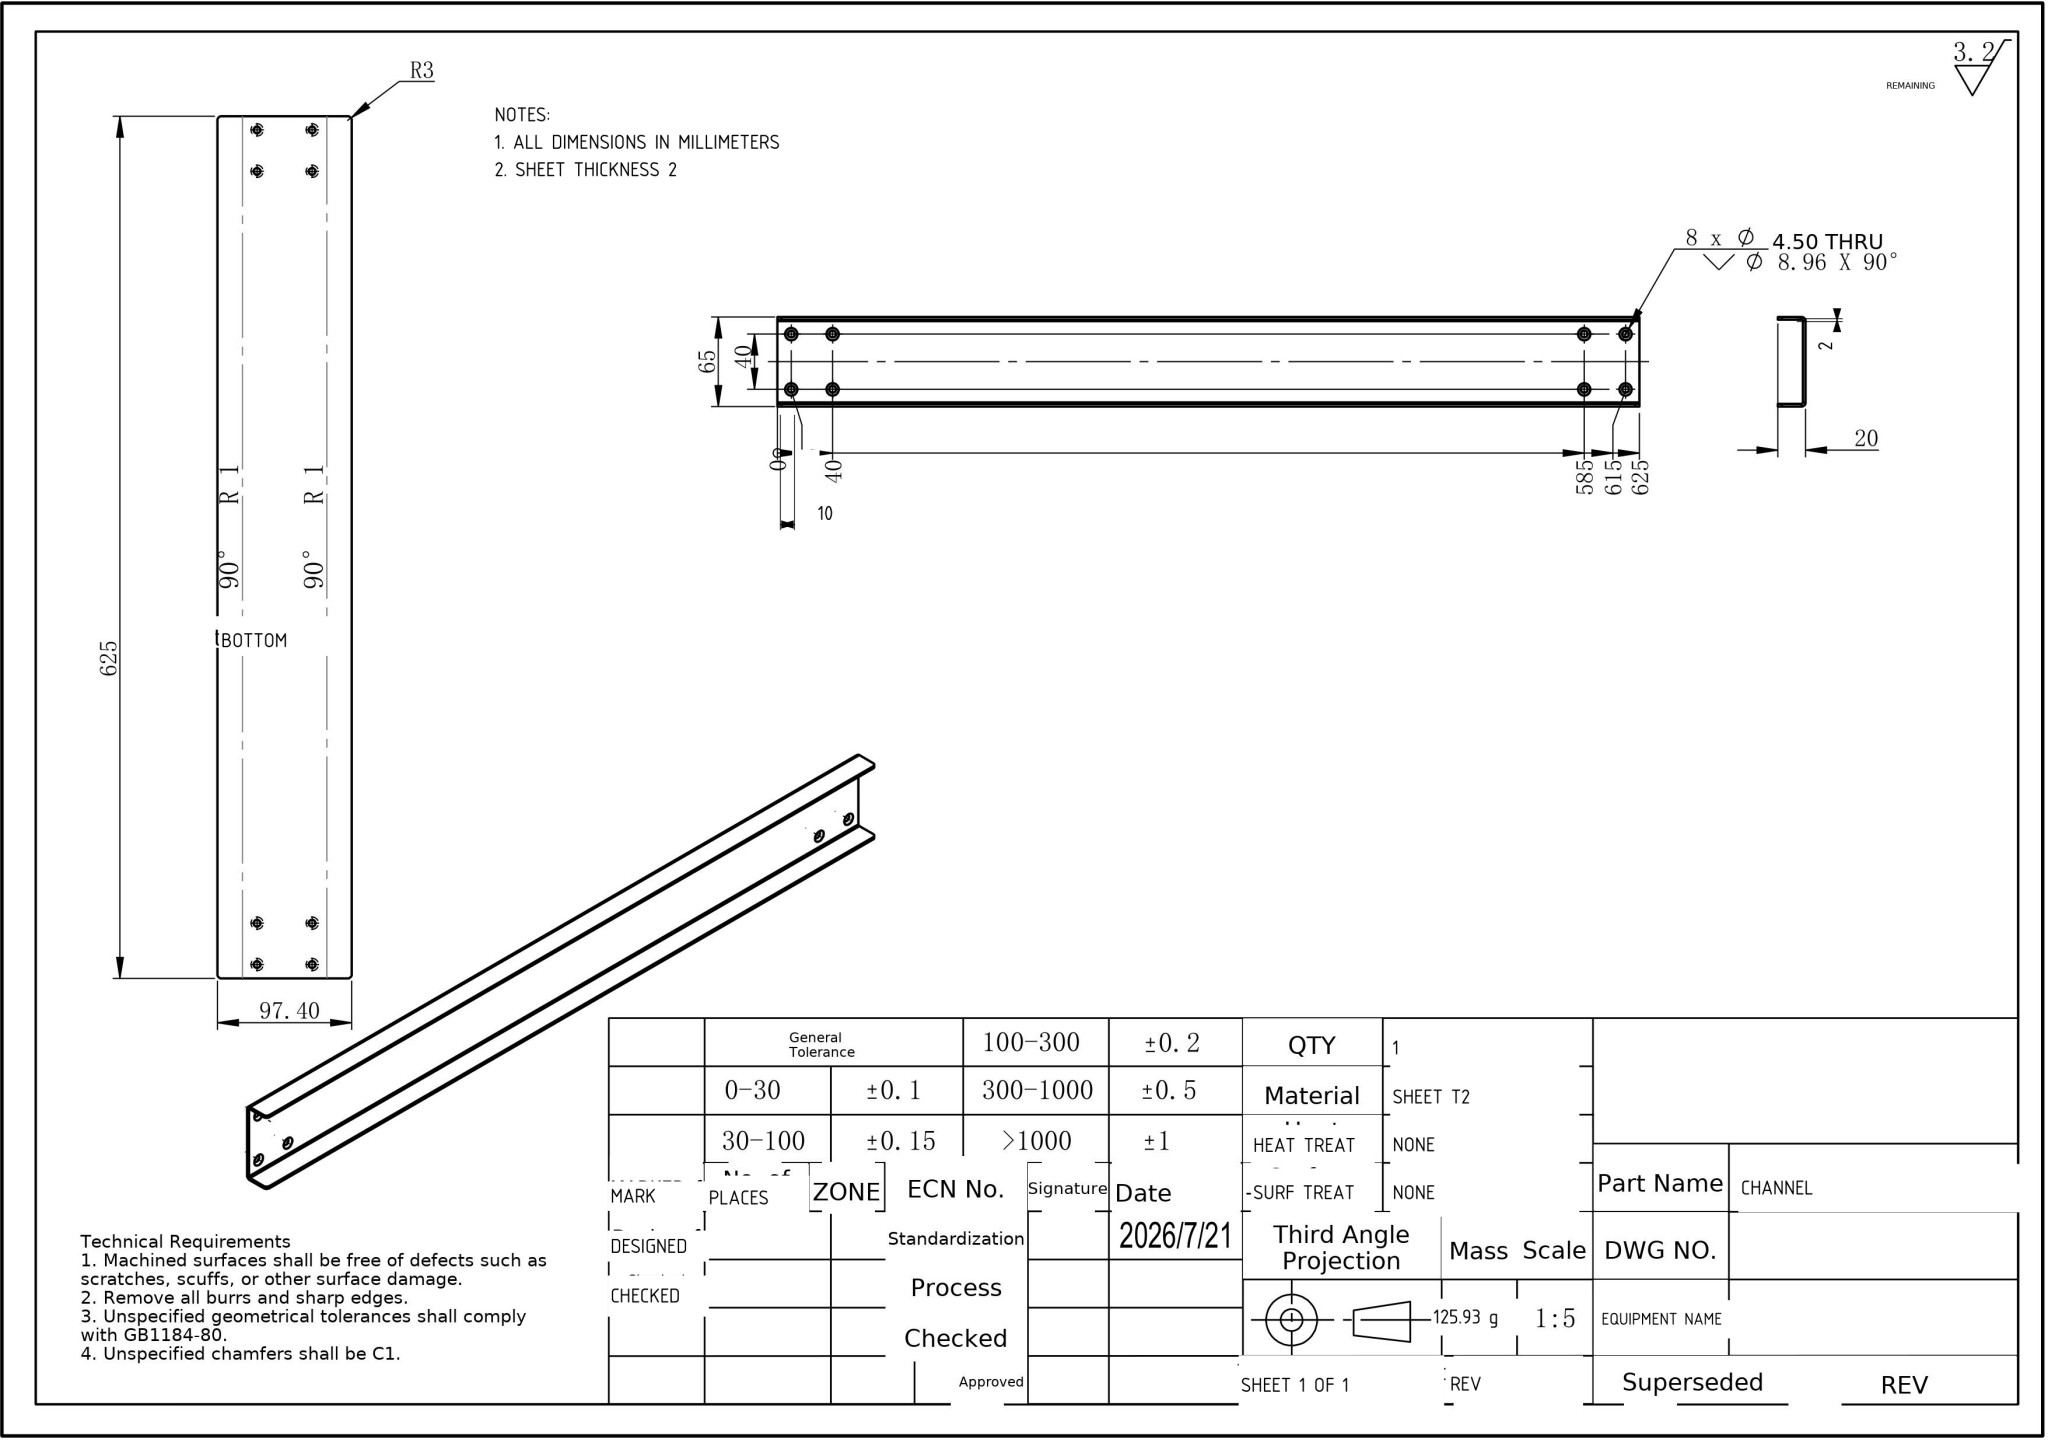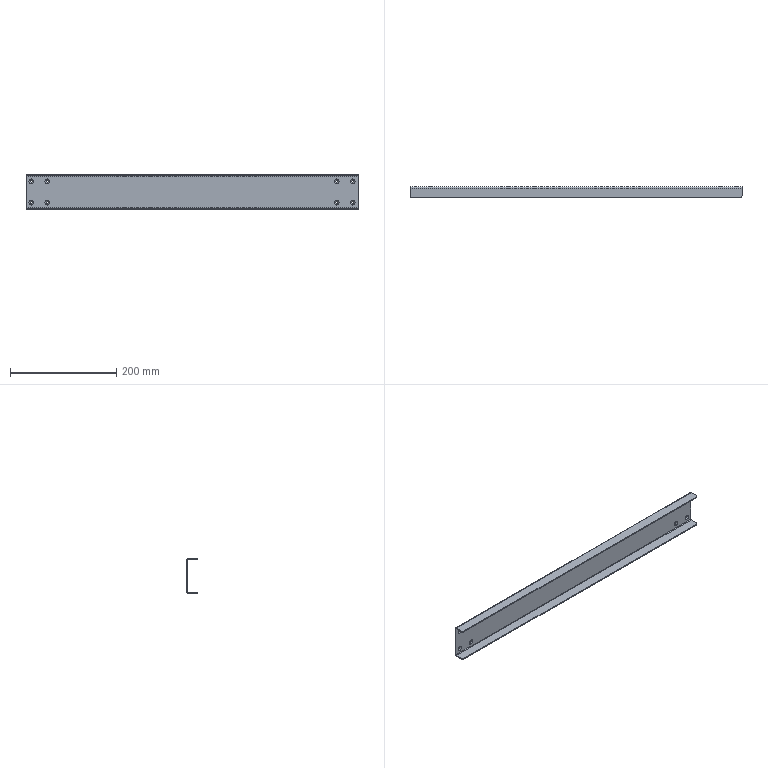Part | NX | mm | 1 solid | 42 faces | box 625 x 20 x 65 mm | volume 123463 mm3 | plane 18 | cone 16 | cylinder 8 | commonest cylinder face diameters 6 x6 2 x2